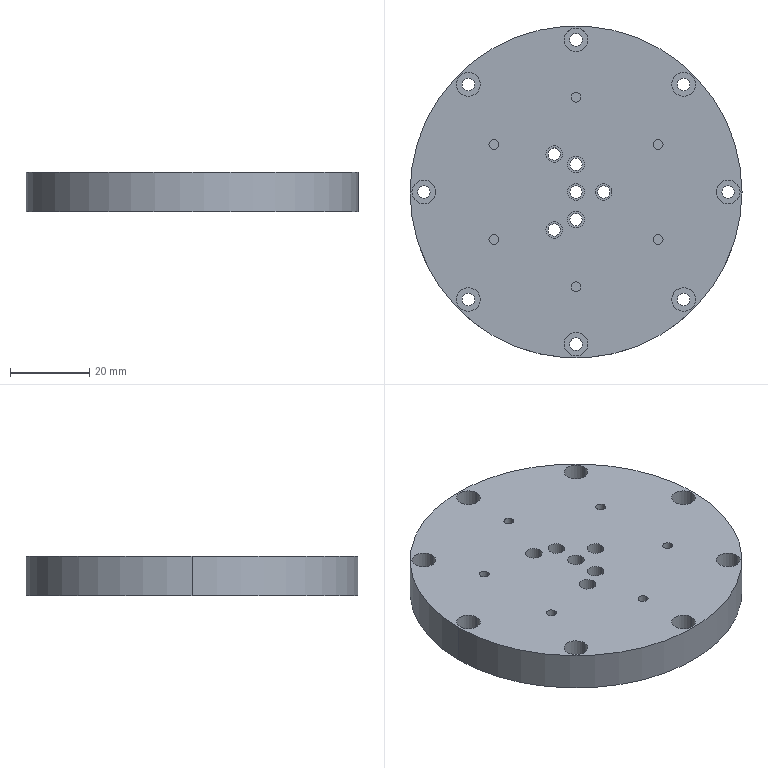CAM job | Mastercam | mm | 4 operations | part box 84 x 84 x 10
1. Contour (Ramp) | 4 - 4 平铣刀
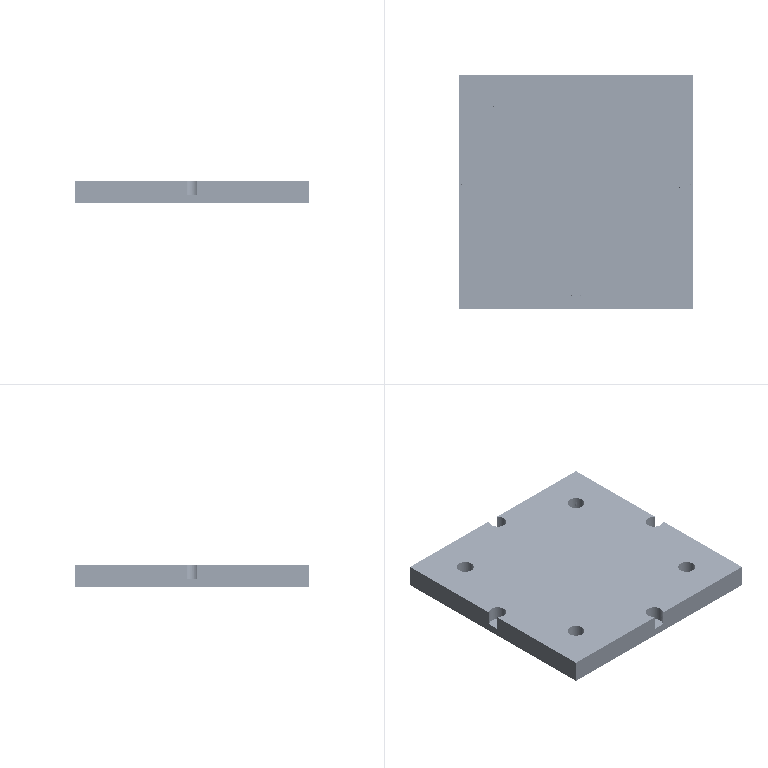2. Contour (2D) | 4 - 4 平铣刀
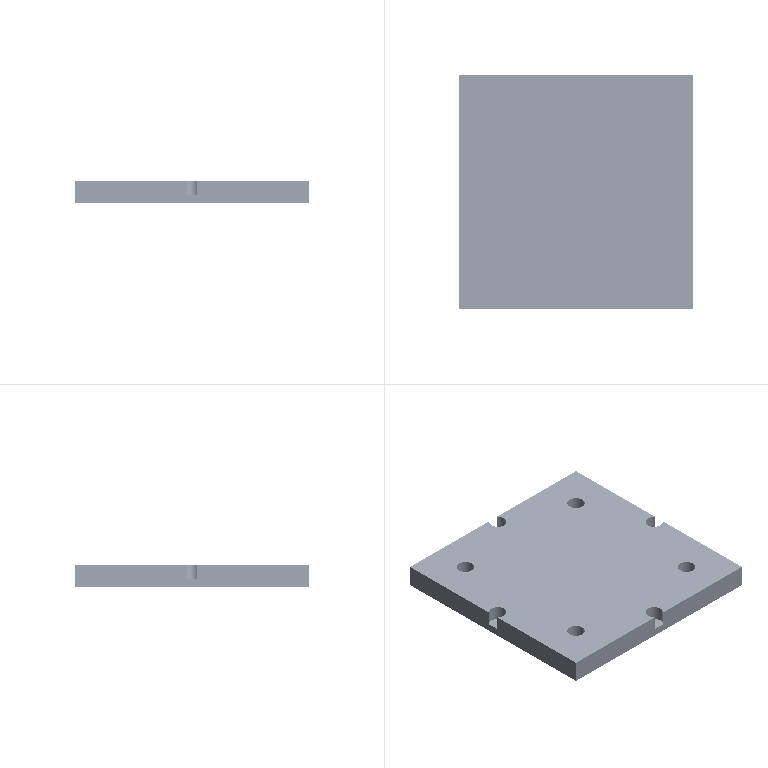3. Drill/Counterbore | 7 - 4 倒角刀
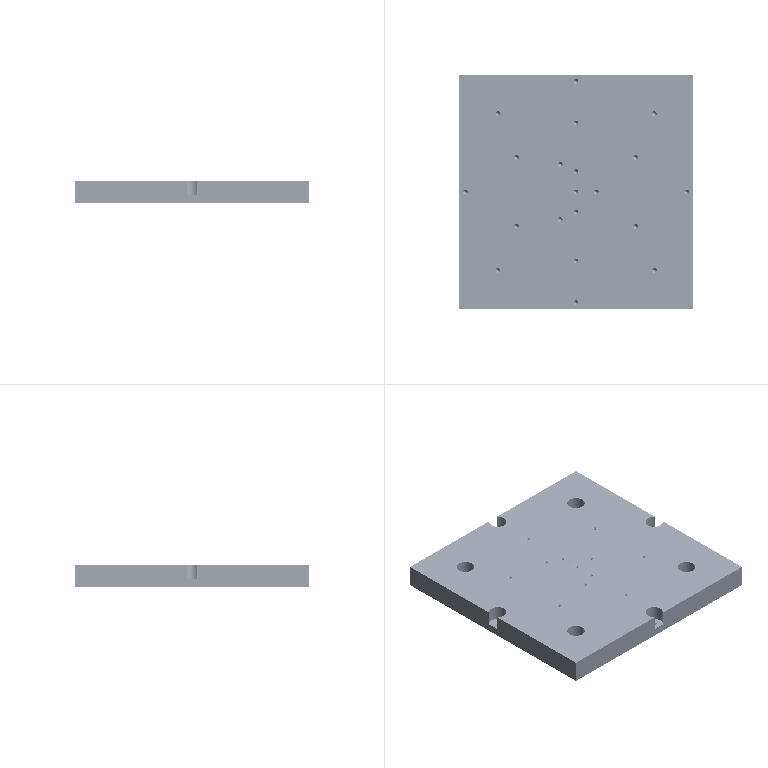4. Contour (2D chamfer) | 7 - 4 倒角刀